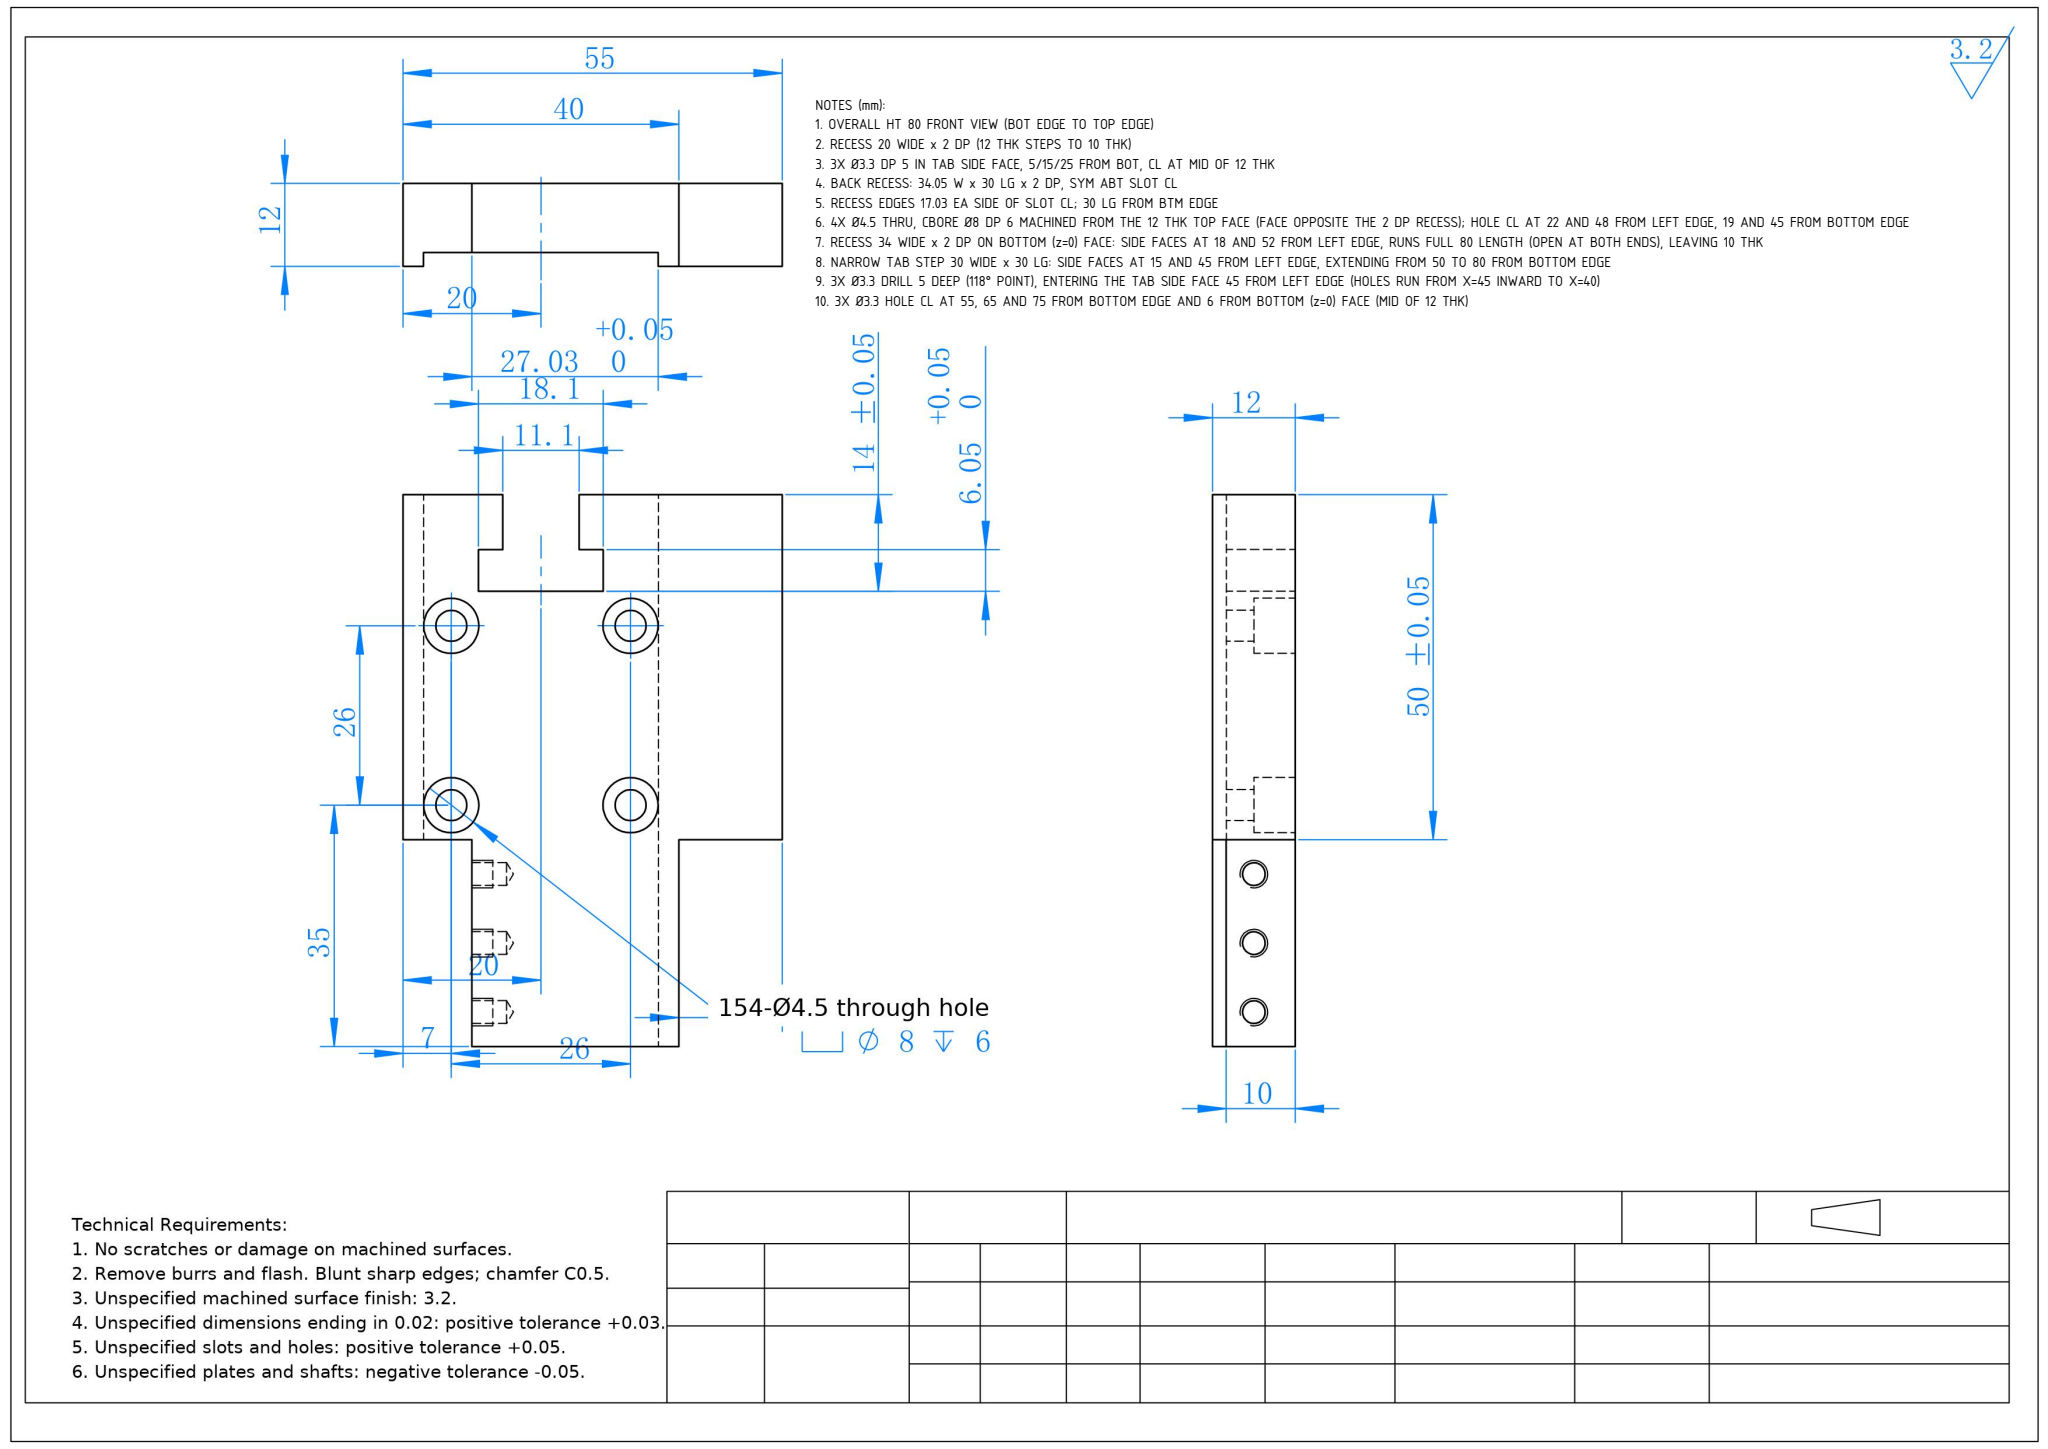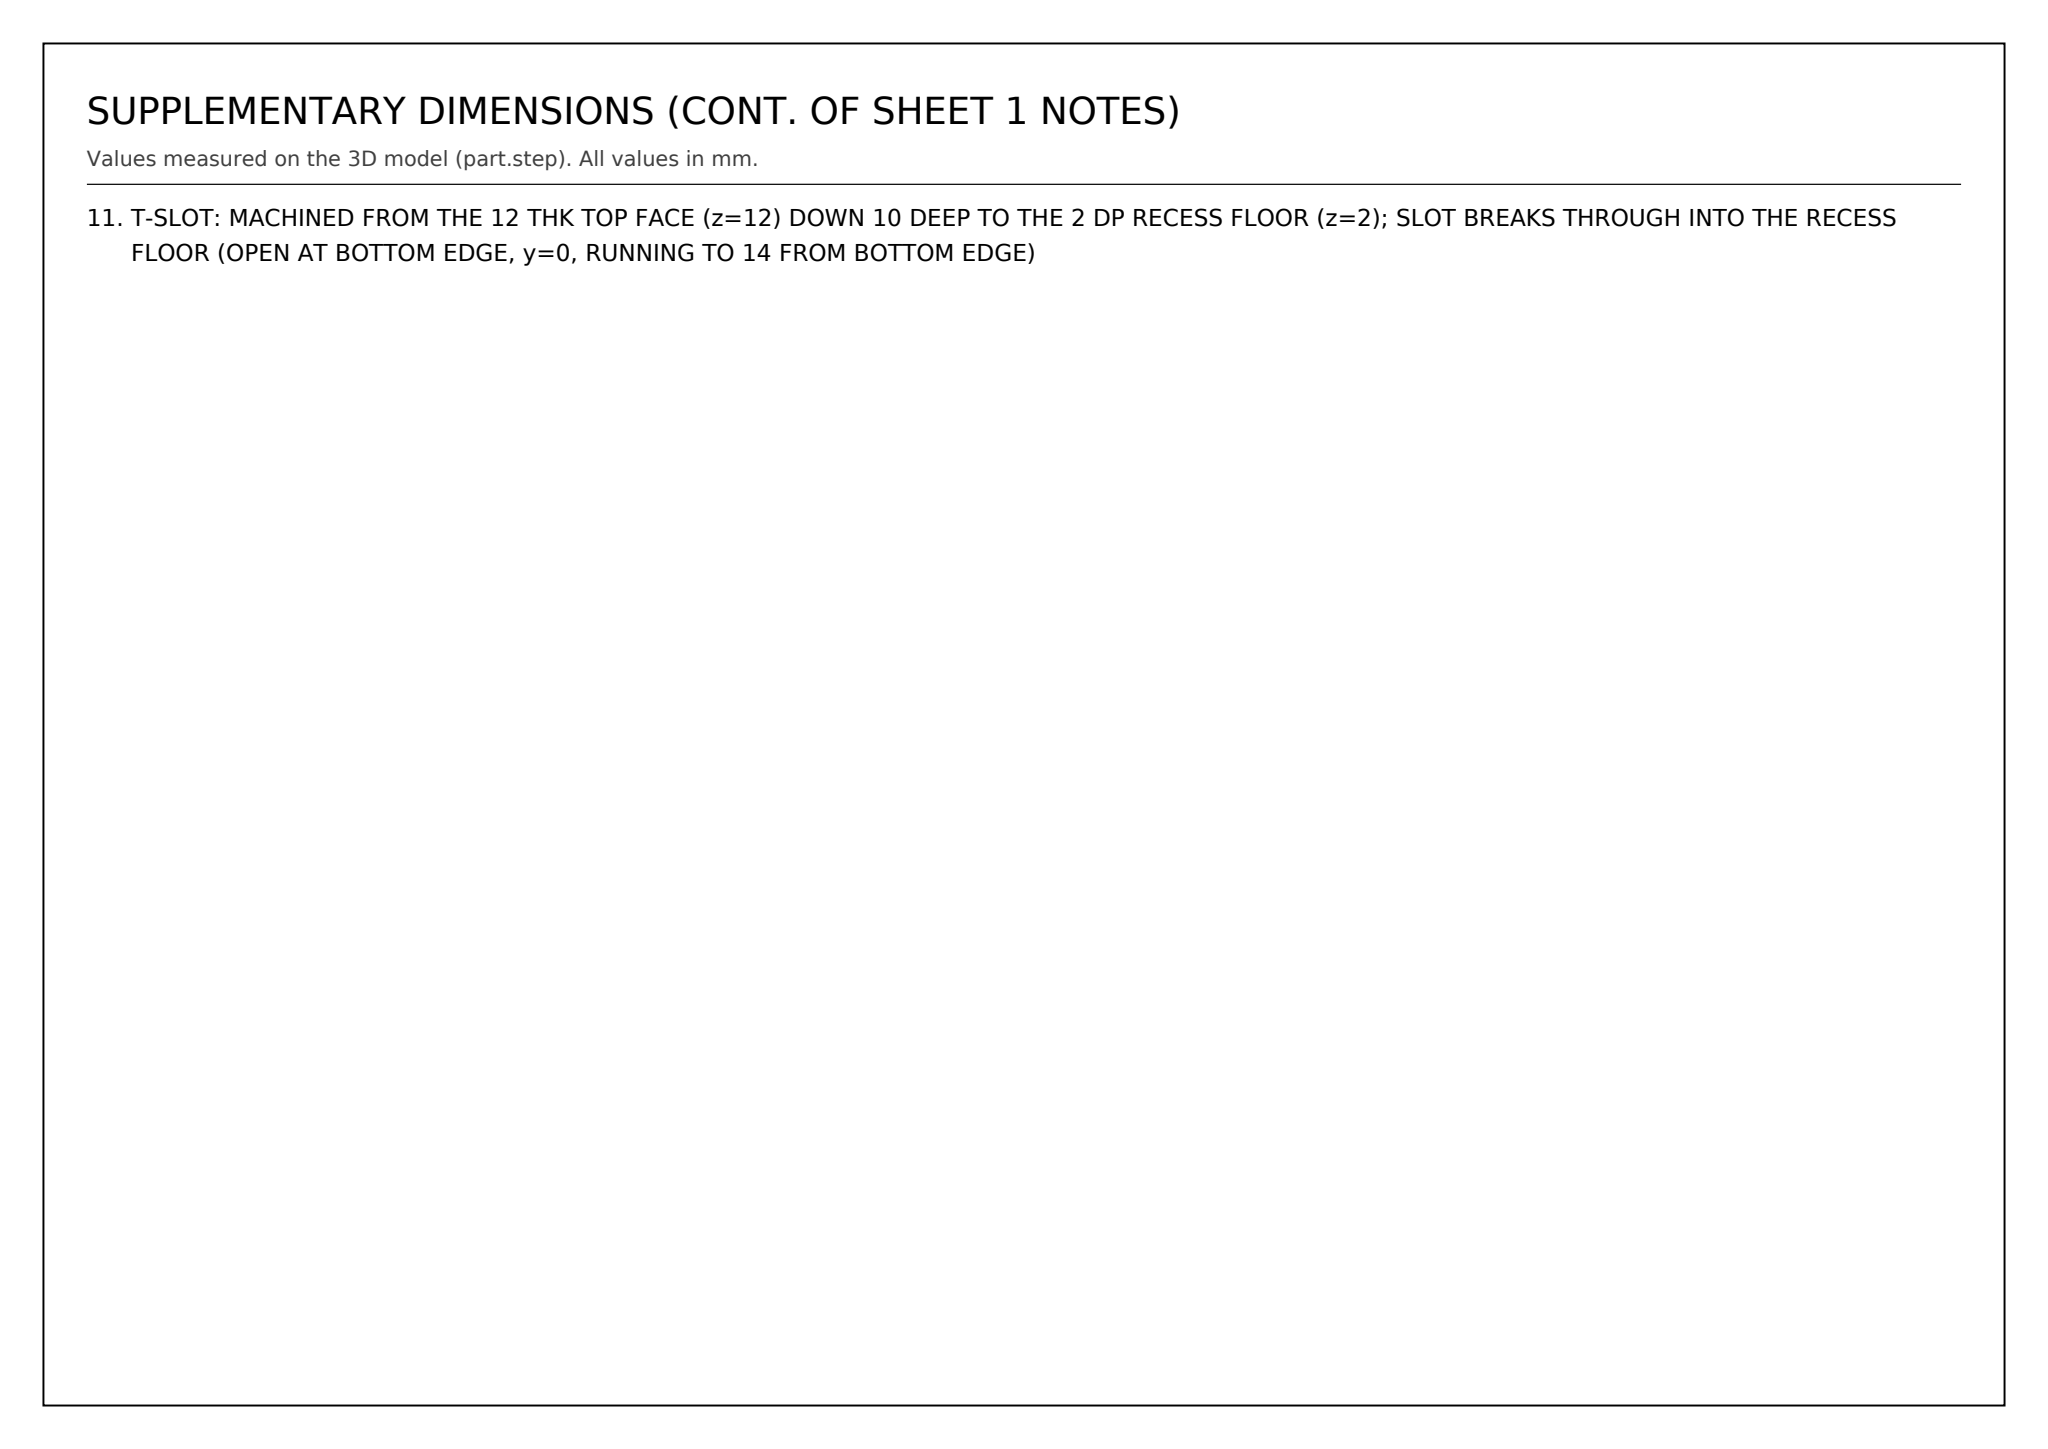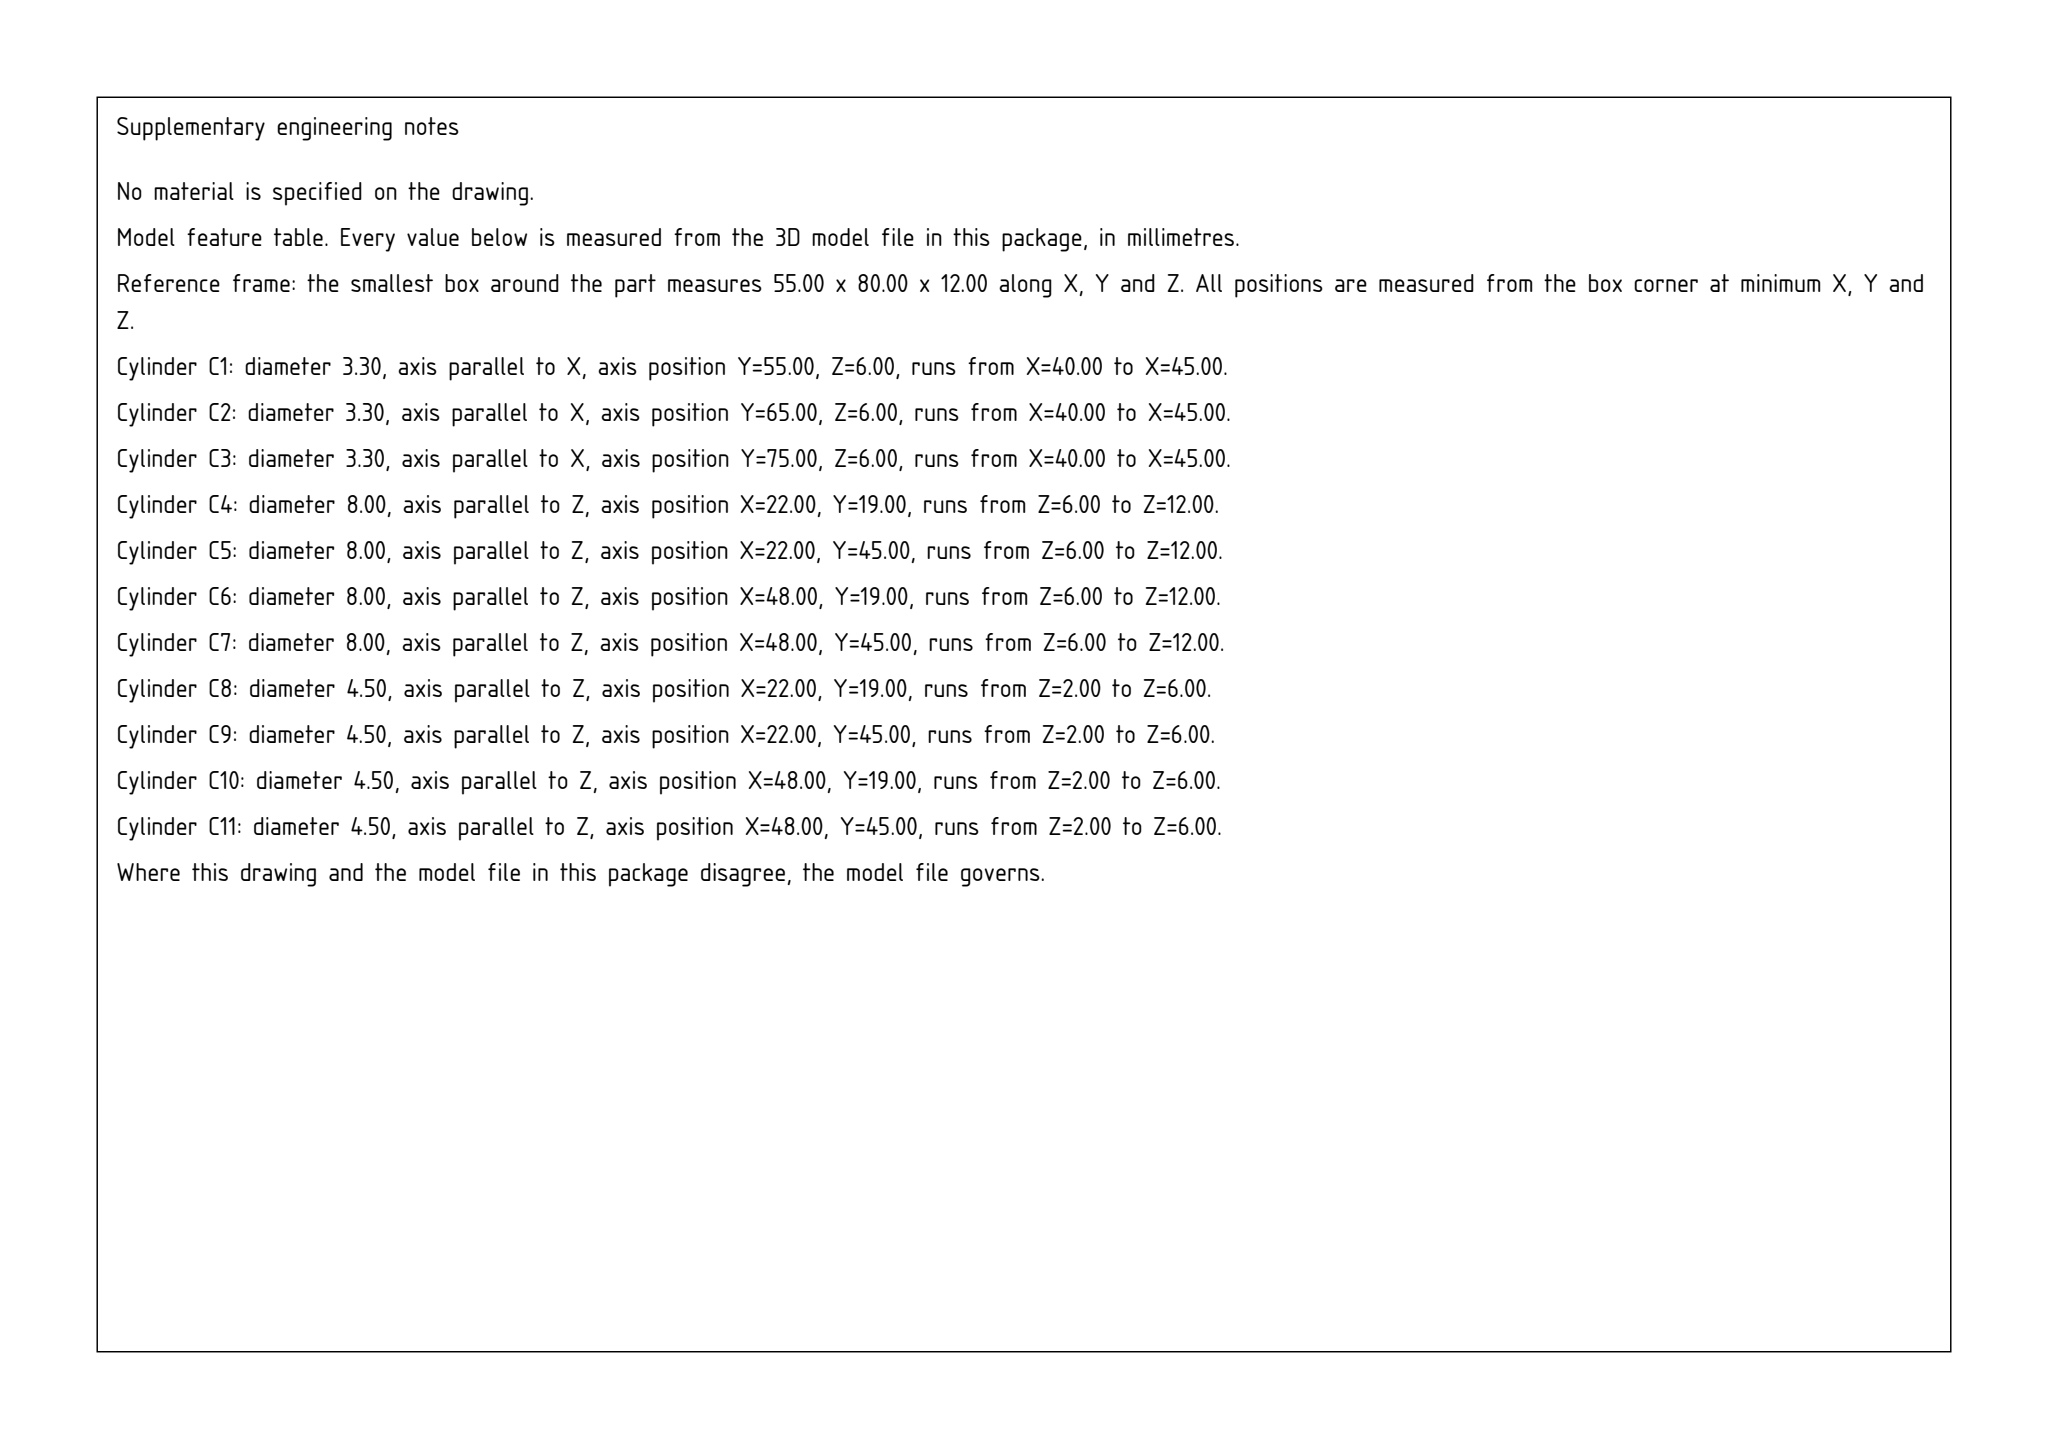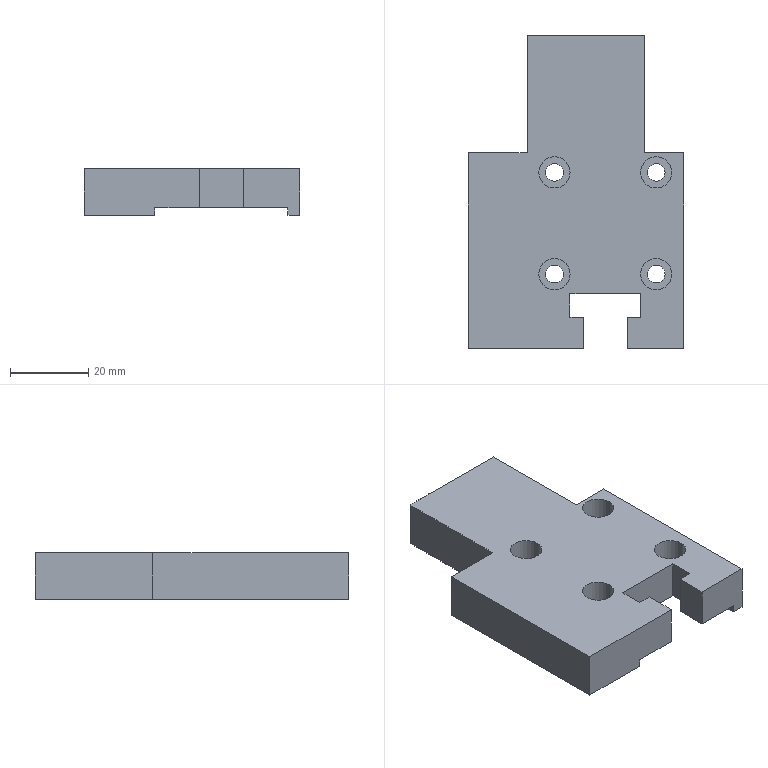Part | SolidWorks | mm | 1 solid | 54 faces | box 55 x 80 x 12 mm | volume 35198 mm3 | plane 26 | cylinder 22 | cone 6 | commonest cylinder face diameters 8 x8 4.5 x8 3.3 x6
Drawing notes:
OVERALL HT 80 FRONT VIEW (BOT EDGE TO TOP EDGE) | from the solid: bbox_xyz Y = 80.0; planes y=0.0 and y=80.0
RECESS 20 WIDE x 2 DP (12 THK STEPS TO 10 THK) | from the solid: z planes 0.0 and 2.0 step floor; side view 12 thk to 10 thk = 2 deep
3X Ø3.3 DP 5 IN TAB SIDE FACE, 5/15/25 FROM BOT, CL AT MID OF 12 THK | from the solid: cyl Ø3.3 axis x at y=55/65/75 (=25/15/5 from y=80 bot edge), z=6 mid of 12 thk, L=5; cones 118° ref Ø3.3
BACK RECESS: 34.05 W x 30 LG x 2 DP, SYM ABT SLOT CL | from the solid: z planes 0 & 2 (2 deep); x planes 17.98 & 52.03 (34.05 wide, mid 35.0 = slot CL from x25.95/44.05 & 29.45/40.55); y 50 to 80 (30 long)
RECESS EDGES 17.03 EA SIDE OF SLOT CL; 30 LG FROM BTM EDGE | from the solid: x planes 17.98 & 52.03 about slot CL x=35.0 (34.05/2=17.03); y plane 50.0 to bbox y 80.0
4X Ø4.5 THRU, CBORE Ø8 DP 6 MACHINED FROM THE 12 THK TOP FACE (FACE OPPOSITE THE 2 DP RECESS); HOLE CL AT 22 AND 48 FROM LEFT EDGE, 19 AND 45 FROM BOTTOM EDGE | from the solid: cylinders: Ø4.5 axis z at (22,19),(22,45),(48,19),(48,45) from z=2 to 6; Ø8 axis z same centers from z=6 to 12 (top face z=12)
RECESS 34 WIDE x 2 DP ON BOTTOM (z=0) FACE: SIDE FACES AT 18 AND 52 FROM LEFT EDGE, RUNS FULL 80 LENGTH (OPEN AT BOTH ENDS), LEAVING 10 THK | from the solid: plane z=2 extent x[18,52], y[0,80]; plane z=0 only at x[0,18] y[0,80] and x[52,55] y[0,50]; planes x=18 and x=52 of height 2
NARROW TAB STEP 30 WIDE x 30 LG: SIDE FACES AT 15 AND 45 FROM LEFT EDGE, EXTENDING FROM 50 TO 80 FROM BOTTOM EDGE | from the solid: planes x=15.0 and x=45.0 with extent y[50,80]; planes y=50 at x[0,15] and x[45,55]; plane y=80 at x[15,45]
3X Ø3.3 DRILL 5 DEEP (118° POINT), ENTERING THE TAB SIDE FACE 45 FROM LEFT EDGE (HOLES RUN FROM X=45 INWARD TO X=40) | from the solid: cylinders: 3X hole/bore dia 3.3, axis x, from 40.0 to 45.0; axis_planes x=45.0 extent y[50,80] z[2,12] (tab side face); cones 118.0 ref_dia 3.3
3X Ø3.3 HOLE CL AT 55, 65 AND 75 FROM BOTTOM EDGE AND 6 FROM BOTTOM (z=0) FACE (MID OF 12 THK) | from the solid: cylinders: hole/bore 3.3 axis x at [null,55.0,6.0], [null,65.0,6.0], [null,75.0,6.0]
T-SLOT: MACHINED FROM THE 12 THK TOP FACE (z=12) DOWN 10 DEEP TO THE 2 DP RECESS FLOOR (z=2); SLOT BREAKS THROUGH INTO THE RECESS FLOOR (OPEN AT BOTTOM EDGE, y=0, RUNNING TO 14 FROM BOTTOM EDGE) | from the solid: axis_planes x=29.5 and x=40.5 (y 0-8) and x=25.9/44.1 (y 8-14) all with z extent [2.0,12.0]; z=12.0 top face and z=2.0 recess floor (x 18-52, y 0-80)
build123d program:
from build123d import *

# Parameters (mm, degrees)
SKETCH1_W                                       = 40
SKETCH1_H                                       = 80
BOSS_EXTRUDE1_DEPTH                             = 12
CUT_EXTRUDE2_DEPTH                              = 47.303
SKETCH15_W                                      = 34.05
SKETCH15_H                                      = 80
CUT_EXTRUDE4_DEPTH                              = 2
M4_HEX_SOCKET_HEAD_CAP_SCREW_CBORE1_D           = 4.5
M4_HEX_SOCKET_HEAD_CAP_SCREW_CBORE1_CBORE_D     = 8
M4_HEX_SOCKET_HEAD_CAP_SCREW_CBORE1_CBORE_DEPTH = 6
SKETCH36_W                                      = 15
SKETCH36_H                                      = 50
BOSS_EXTRUDE3_DEPTH                             = 12
M4_TAPPED_HOLE2_D                               = 3.3
M4_TAPPED_HOLE2_DEPTH                           = 15
M4_TAPPED_HOLE2_TIP                             = 0.9914
SKETCH40_W                                      = 12
SKETCH40_H                                      = 30
CUT_EXTRUDE5_DEPTH                              = 10


with BuildPart() as part:
    # Sketch1 → Boss-Extrude1 (new body)
    with BuildSketch(Plane.XY):
        Rectangle(SKETCH1_W, SKETCH1_H)
    extrude(amount=BOSS_EXTRUDE1_DEPTH)

    # Sketch5 → Cut-Extrude2 (cut, through all)
    with BuildSketch(Plane.XY.offset(12)):
        Polygon((5.55, -32.05), (9.05, -32.05), (9.05, -26), (-9.05, -26), (-9.05, -32.05), (-5.55, -32.05), (-5.55, -40), (5.55, -40), align=None)
    extrude(amount=-CUT_EXTRUDE2_DEPTH, mode=Mode.SUBTRACT)

    # Sketch15 → Cut-Extrude4 (cut)
    with BuildSketch(Plane(origin=(0, 0, 0), x_dir=(-1, 0, 0), z_dir=(0, 0, -1))):
        Rectangle(SKETCH15_W, SKETCH15_H)
    extrude(amount=-CUT_EXTRUDE4_DEPTH, mode=Mode.SUBTRACT)

    # M4 Hex Socket Head Cap Screw CBORE1 (through all)
    with Locations(Plane.XY.offset(12)):
        with Locations((-13, -21), (13, -21), (-13, 5), (13, 5)):
            CounterBoreHole(M4_HEX_SOCKET_HEAD_CAP_SCREW_CBORE1_D / 2, M4_HEX_SOCKET_HEAD_CAP_SCREW_CBORE1_CBORE_D / 2, M4_HEX_SOCKET_HEAD_CAP_SCREW_CBORE1_CBORE_DEPTH)

    # Sketch36 → Boss-Extrude3 (add)
    with BuildSketch(Plane.XY.offset(12)):
        with Locations((-27.5, -15)):
            Rectangle(SKETCH36_W, SKETCH36_H)
    extrude(amount=-BOSS_EXTRUDE3_DEPTH)

    # M4 Tapped Hole2
    with Locations(Plane(origin=(20, 0, 0), x_dir=(0, 0, -1), z_dir=(1, 0, 0))):
        with Locations((-6, 15), (-6, 25), (-6, 35)):
            Hole(M4_TAPPED_HOLE2_D / 2, depth=M4_TAPPED_HOLE2_DEPTH)
            with Locations((0, 0, -(M4_TAPPED_HOLE2_DEPTH + M4_TAPPED_HOLE2_TIP / 2))):  # 118° drill point
                Cone(0, M4_TAPPED_HOLE2_D / 2, M4_TAPPED_HOLE2_TIP, mode=Mode.SUBTRACT)

    # Sketch40 → Cut-Extrude5 (cut)
    with BuildSketch(Plane(origin=(20, 0, 0), x_dir=(0, 0, -1), z_dir=(1, 0, 0))):
        with Locations((-6, 25)):
            Rectangle(SKETCH40_W, SKETCH40_H)
    extrude(amount=-CUT_EXTRUDE5_DEPTH, mode=Mode.SUBTRACT)


solid = part.part